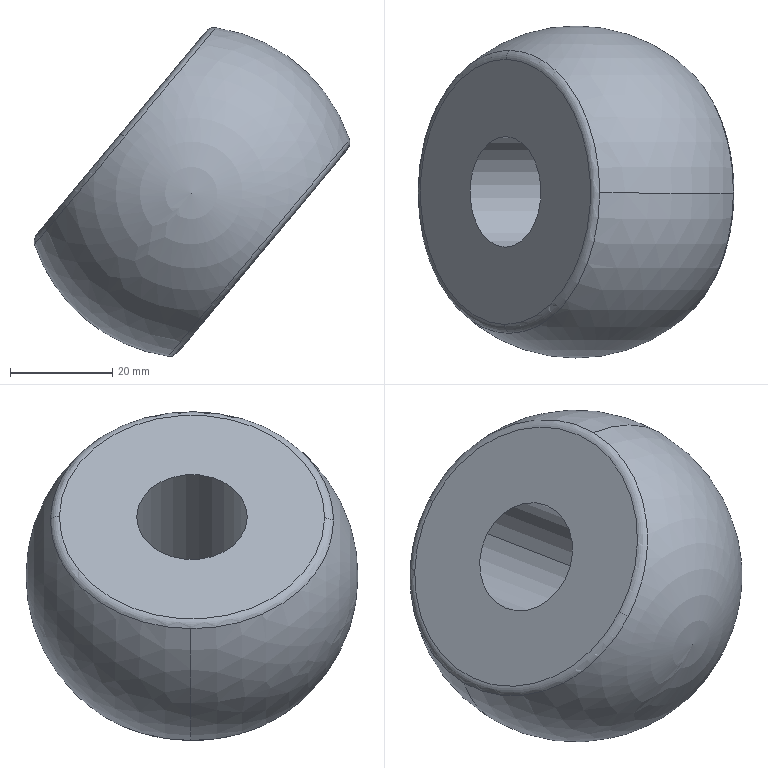Component | SolidWorks | 30-01A-1_Wheel-322-1_CJH65-322-1_CJH65wheel-322-1 | 1 solid | 10 faces | box 61.85 x 65 x 64.37 mm | volume 93907 mm3 | torus 4 | sphere 2 | cylinder 2 | plane 2 | commonest cylinder face diameters 21.667 x2
build123d program:
from build123d import *


with BuildPart() as part:
    # Sketch1 → Revolve1 (revolve)
    with BuildSketch(Plane.XY, mode=Mode.PRIVATE) as revolve1_sk:
        with BuildLine():
            Line((-18, 10.833), (18, 10.833))
            Line((18, 10.833), (18, 25.966))
            ThreePointArc((18, 25.966), (17.746, 26.941), (17.049, 27.669))
            ThreePointArc((17.049, 27.669), (0, 32.5), (-17.049, 27.669))
            ThreePointArc((-17.049, 27.669), (-17.746, 26.941), (-18, 25.966))
            Line((-18, 25.966), (-18, 10.833))
        make_face()
    revolve(revolve1_sk.sketch.rotate(Axis((50, 0, 0), (-1, 0, 0)), 270), axis=Axis((50, 0, 0), (-1, 0, 0)))


solid = part.part

# Placed as in the assembly
solid = solid.moved(Location((177.3, -622.345, -91.473), (-89.646, 0.2952, -140.136)))
STEP:
#1=CARTESIAN_POINT('',(5.767,-24.493,-4.007));
#2=VERTEX_POINT('',#1);
#3=CARTESIAN_POINT('',(6.46,-25.591,-3.178));
#4=VERTEX_POINT('',#3);
#5=CARTESIAN_POINT('',(6.465,-24.502,-3.171));
#6=DIRECTION('',(-0.7676,0.,0.641));
#7=DIRECTION('',(0.00514,1.,0.006155));
#8=AXIS2_PLACEMENT_3D('',#5,#6,#7);
#9=CIRCLE('',#8,1.089);
#10=EDGE_CURVE('',#2,#4,#9,.T.);
#11=ORIENTED_EDGE('',*,*,#10,.T.);
#12=CARTESIAN_POINT('',(6.431,-25.524,-3.153));
#13=VERTEX_POINT('',#12);
#14=CARTESIAN_POINT('',(6.492,-25.524,-3.204));
#15=DIRECTION('',(-0.641,0.008019,-0.7675));
#16=DIRECTION('',(-0.7676,0.,0.641));
#17=AXIS2_PLACEMENT_3D('',#14,#15,#16);
#18=CIRCLE('',#17,0.07874);
#19=EDGE_CURVE('',#4,#13,#18,.T.);
#20=ORIENTED_EDGE('',*,*,#19,.T.);
#21=CARTESIAN_POINT('',(6.442,-23.479,-3.141));
#22=VERTEX_POINT('',#21);
#23=CARTESIAN_POINT('',(6.436,-24.502,-3.147));
#24=DIRECTION('',(-0.7676,0.,0.641));
#25=DIRECTION('',(0.00514,1.,0.006155));
#26=AXIS2_PLACEMENT_3D('',#23,#24,#25);
#27=CIRCLE('',#26,1.022);
#28=EDGE_CURVE('',#22,#13,#27,.T.);
#29=ORIENTED_EDGE('',*,*,#28,.F.);
#30=CARTESIAN_POINT('',(6.471,-23.412,-3.164));
#31=VERTEX_POINT('',#30);
#32=CARTESIAN_POINT('',(6.502,-23.479,-3.191));
#33=DIRECTION('',(0.641,-0.008019,0.7675));
#34=DIRECTION('',(0.7676,0.,-0.641));
#35=AXIS2_PLACEMENT_3D('',#32,#33,#34);
#36=CIRCLE('',#35,0.07874);
#37=EDGE_CURVE('',#31,#22,#36,.T.);
#38=ORIENTED_EDGE('',*,*,#37,.F.);
#39=CARTESIAN_POINT('',(6.465,-24.502,-3.171));
#40=DIRECTION('',(-0.7676,0.,0.641));
#41=DIRECTION('',(0.00514,1.,0.006155));
#42=AXIS2_PLACEMENT_3D('',#39,#40,#41);
#43=CIRCLE('',#42,1.089);
#44=EDGE_CURVE('',#31,#2,#43,.T.);
#45=ORIENTED_EDGE('',*,*,#44,.T.);
#46=EDGE_LOOP('',(#11,#20,#29,#38,#45));
#47=FACE_OUTER_BOUND('',#46,.T.);
#48=CARTESIAN_POINT('',(6.497,-24.502,-3.198));
#49=DIRECTION('',(-0.7676,0.,0.641));
#50=DIRECTION('',(0.00514,1.,0.006155));
#51=AXIS2_PLACEMENT_3D('',#48,#49,#50);
#52=TOROIDAL_SURFACE('',#51,1.022,0.07874);
#53=ADVANCED_FACE('',(#47),#52,.T.);
#54=CARTESIAN_POINT('',(7.49,-25.591,-4.038));
#55=VERTEX_POINT('',#54);
#56=CARTESIAN_POINT('',(8.194,-24.51,-3.195));
#57=VERTEX_POINT('',#56);
#58=CARTESIAN_POINT('',(7.496,-24.502,-4.032));
#59=DIRECTION('',(-0.7676,0.,0.641));
#60=DIRECTION('',(0.00514,1.,0.006155));
#61=AXIS2_PLACEMENT_3D('',#58,#59,#60);
#62=CIRCLE('',#61,1.089);
#63=EDGE_CURVE('',#55,#57,#62,.T.);
#64=ORIENTED_EDGE('',*,*,#63,.T.);
#65=CARTESIAN_POINT('',(7.163,-24.51,-2.335));
#66=VERTEX_POINT('',#65);
#67=CARTESIAN_POINT('',(6.98,-24.502,-3.601));
#68=DIRECTION('',(-0.00514,-1.,-0.006155));
#69=DIRECTION('',(0.,0.006155,-1.));
#70=AXIS2_PLACEMENT_3D('',#67,#68,#69);
#71=CIRCLE('',#70,1.28);
#72=EDGE_CURVE('',#57,#66,#71,.T.);
#73=ORIENTED_EDGE('',*,*,#72,.T.);
#74=CARTESIAN_POINT('',(6.465,-24.502,-3.171));
#75=DIRECTION('',(-0.7676,0.,0.641));
#76=DIRECTION('',(0.00514,1.,0.006155));
#77=AXIS2_PLACEMENT_3D('',#74,#75,#76);
#78=CIRCLE('',#77,1.089);
#79=EDGE_CURVE('',#4,#66,#78,.T.);
#80=ORIENTED_EDGE('',*,*,#79,.F.);
#81=ORIENTED_EDGE('',*,*,#10,.F.);
#82=CARTESIAN_POINT('',(6.797,-24.493,-4.868));
#83=VERTEX_POINT('',#82);
#84=CARTESIAN_POINT('',(6.98,-24.502,-3.601));
#85=DIRECTION('',(0.00514,1.,0.006155));
#86=DIRECTION('',(0.,-0.006155,1.));
#87=AXIS2_PLACEMENT_3D('',#84,#85,#86);
#88=CIRCLE('',#87,1.28);
#89=EDGE_CURVE('',#83,#2,#88,.T.);
#90=ORIENTED_EDGE('',*,*,#89,.F.);
#91=CARTESIAN_POINT('',(7.496,-24.502,-4.032));
#92=DIRECTION('',(-0.7676,0.,0.641));
#93=DIRECTION('',(0.00514,1.,0.006155));
#94=AXIS2_PLACEMENT_3D('',#91,#92,#93);
#95=CIRCLE('',#94,1.089);
#96=EDGE_CURVE('',#83,#55,#95,.T.);
#97=ORIENTED_EDGE('',*,*,#96,.T.);
#98=EDGE_LOOP('',(#64,#73,#80,#81,#90,#97));
#99=FACE_OUTER_BOUND('',#98,.T.);
#100=CARTESIAN_POINT('',(6.98,-24.502,-3.601));
#101=DIRECTION('',(-0.00514,-1.,-0.006155));
#102=DIRECTION('',(-0.641,0.008019,-0.7675));
#103=AXIS2_PLACEMENT_3D('',#100,#101,#102);
#104=SPHERICAL_SURFACE('',#103,1.28);
#105=ADVANCED_FACE('',(#99),#104,.T.);
#106=CARTESIAN_POINT('',(7.529,-23.479,-4.049));
#107=VERTEX_POINT('',#106);
#108=CARTESIAN_POINT('',(7.519,-25.524,-4.062));
#109=VERTEX_POINT('',#108);
#110=CARTESIAN_POINT('',(7.524,-24.502,-4.056));
#111=DIRECTION('',(-0.7676,0.,0.641));
#112=DIRECTION('',(0.00514,1.,0.006155));
#113=AXIS2_PLACEMENT_3D('',#110,#111,#112);
#114=CIRCLE('',#113,1.022);
#115=EDGE_CURVE('',#107,#109,#114,.T.);
#116=ORIENTED_EDGE('',*,*,#115,.T.);
#117=CARTESIAN_POINT('',(7.459,-25.524,-4.011));
#118=DIRECTION('',(-0.641,0.008019,-0.7675));
#119=DIRECTION('',(-0.7676,0.,0.641));
#120=AXIS2_PLACEMENT_3D('',#117,#118,#119);
#121=CIRCLE('',#120,0.07874);
#122=EDGE_CURVE('',#109,#55,#121,.T.);
#123=ORIENTED_EDGE('',*,*,#122,.T.);
#124=ORIENTED_EDGE('',*,*,#96,.F.);
#125=CARTESIAN_POINT('',(7.501,-23.412,-4.025));
#126=VERTEX_POINT('',#125);
#127=CARTESIAN_POINT('',(7.496,-24.502,-4.032));
#128=DIRECTION('',(-0.7676,0.,0.641));
#129=DIRECTION('',(0.00514,1.,0.006155));
#130=AXIS2_PLACEMENT_3D('',#127,#128,#129);
#131=CIRCLE('',#130,1.089);
#132=EDGE_CURVE('',#126,#83,#131,.T.);
#133=ORIENTED_EDGE('',*,*,#132,.F.);
#134=CARTESIAN_POINT('',(7.469,-23.479,-3.999));
#135=DIRECTION('',(0.641,-0.008019,0.7675));
#136=DIRECTION('',(0.7676,0.,-0.641));
#137=AXIS2_PLACEMENT_3D('',#134,#135,#136);
#138=CIRCLE('',#137,0.07874);
#139=EDGE_CURVE('',#107,#126,#138,.T.);
#140=ORIENTED_EDGE('',*,*,#139,.F.);
#141=EDGE_LOOP('',(#116,#123,#124,#133,#140));
#142=FACE_OUTER_BOUND('',#141,.T.);
#143=CARTESIAN_POINT('',(7.464,-24.502,-4.005));
#144=DIRECTION('',(-0.7676,0.,0.641));
#145=DIRECTION('',(0.00514,1.,0.006155));
#146=AXIS2_PLACEMENT_3D('',#143,#144,#145);
#147=TOROIDAL_SURFACE('',#146,1.022,0.07874);
#148=ADVANCED_FACE('',(#142),#147,.T.);
#149=CARTESIAN_POINT('',(7.522,-24.928,-4.058));
#150=VERTEX_POINT('',#149);
#151=CARTESIAN_POINT('',(7.526,-24.075,-4.053));
#152=VERTEX_POINT('',#151);
#153=CARTESIAN_POINT('',(7.524,-24.502,-4.056));
#154=DIRECTION('',(-0.7676,0.,0.641));
#155=DIRECTION('',(0.00514,1.,0.006155));
#156=AXIS2_PLACEMENT_3D('',#153,#154,#155);
#157=CIRCLE('',#156,0.4265);
#158=EDGE_CURVE('',#150,#152,#157,.T.);
#159=ORIENTED_EDGE('',*,*,#158,.F.);
#160=CARTESIAN_POINT('',(6.434,-24.928,-3.15));
#161=VERTEX_POINT('',#160);
#162=CARTESIAN_POINT('',(8.489,-24.928,-4.866));
#163=DIRECTION('',(-0.7676,0.,0.641));
#164=VECTOR('',#163,39.37);
#165=LINE('',#162,#164);
#166=EDGE_CURVE('',#150,#161,#165,.T.);
#167=ORIENTED_EDGE('',*,*,#166,.T.);
#168=CARTESIAN_POINT('',(6.439,-24.075,-3.144));
#169=VERTEX_POINT('',#168);
#170=CARTESIAN_POINT('',(6.436,-24.502,-3.147));
#171=DIRECTION('',(-0.7676,0.,0.641));
#172=DIRECTION('',(0.00514,1.,0.006155));
#173=AXIS2_PLACEMENT_3D('',#170,#171,#172);
#174=CIRCLE('',#173,0.4265);
#175=EDGE_CURVE('',#161,#169,#174,.T.);
#176=ORIENTED_EDGE('',*,*,#175,.T.);
#177=CARTESIAN_POINT('',(8.493,-24.075,-4.86));
#178=DIRECTION('',(-0.7676,0.,0.641));
#179=VECTOR('',#178,39.37);
#180=LINE('',#177,#179);
#181=EDGE_CURVE('',#152,#169,#180,.T.);
#182=ORIENTED_EDGE('',*,*,#181,.F.);
#183=EDGE_LOOP('',(#159,#167,#176,#182));
#184=FACE_OUTER_BOUND('',#183,.T.);
#185=CARTESIAN_POINT('',(8.491,-24.502,-4.863));
#186=DIRECTION('',(-0.7676,0.,0.641));
#187=DIRECTION('',(0.00514,1.,0.006155));
#188=AXIS2_PLACEMENT_3D('',#185,#186,#187);
#189=CYLINDRICAL_SURFACE('',#188,0.4265);
#190=ADVANCED_FACE('',(#184),#189,.F.);
#191=CARTESIAN_POINT('',(6.436,-24.502,-3.147));
#192=DIRECTION('',(-0.7676,0.,0.641));
#193=DIRECTION('',(0.00514,1.,0.006155));
#194=AXIS2_PLACEMENT_3D('',#191,#192,#193);
#195=CIRCLE('',#194,0.4265);
#196=EDGE_CURVE('',#169,#161,#195,.T.);
#197=ORIENTED_EDGE('',*,*,#196,.F.);
#198=ORIENTED_EDGE('',*,*,#175,.F.);
#199=EDGE_LOOP('',(#197,#198));
#200=FACE_BOUND('',#199,.T.);
#201=ORIENTED_EDGE('',*,*,#28,.T.);
#202=CARTESIAN_POINT('',(6.436,-24.502,-3.147));
#203=DIRECTION('',(-0.7676,0.,0.641));
#204=DIRECTION('',(0.00514,1.,0.006155));
#205=AXIS2_PLACEMENT_3D('',#202,#203,#204);
#206=CIRCLE('',#205,1.022);
#207=EDGE_CURVE('',#13,#22,#206,.T.);
#208=ORIENTED_EDGE('',*,*,#207,.T.);
#209=EDGE_LOOP('',(#201,#208));
#210=FACE_OUTER_BOUND('',#209,.T.);
#211=CARTESIAN_POINT('',(5.781,-24.494,-3.932));
#212=DIRECTION('',(0.7676,-0.,-0.641));
#213=DIRECTION('',(-0.00514,-1.,-0.006155));
#214=AXIS2_PLACEMENT_3D('',#211,#212,#213);
#215=PLANE('',#214);
#216=ADVANCED_FACE('',(#200,#210),#215,.F.);
#217=ORIENTED_EDGE('',*,*,#166,.F.);
#218=CARTESIAN_POINT('',(7.524,-24.502,-4.056));
#219=DIRECTION('',(-0.7676,0.,0.641));
#220=DIRECTION('',(0.00514,1.,0.006155));
#221=AXIS2_PLACEMENT_3D('',#218,#219,#220);
#222=CIRCLE('',#221,0.4265);
#223=EDGE_CURVE('',#152,#150,#222,.T.);
#224=ORIENTED_EDGE('',*,*,#223,.F.);
#225=ORIENTED_EDGE('',*,*,#181,.T.);
#226=ORIENTED_EDGE('',*,*,#196,.T.);
#227=EDGE_LOOP('',(#217,#224,#225,#226));
#228=FACE_OUTER_BOUND('',#227,.T.);
#229=CARTESIAN_POINT('',(8.491,-24.502,-4.863));
#230=DIRECTION('',(-0.7676,0.,0.641));
#231=DIRECTION('',(0.00514,1.,0.006155));
#232=AXIS2_PLACEMENT_3D('',#229,#230,#231);
#233=CYLINDRICAL_SURFACE('',#232,0.4265);
#234=ADVANCED_FACE('',(#228),#233,.F.);
#235=ORIENTED_EDGE('',*,*,#115,.F.);
#236=CARTESIAN_POINT('',(7.524,-24.502,-4.056));
#237=DIRECTION('',(-0.7676,0.,0.641));
#238=DIRECTION('',(0.00514,1.,0.006155));
#239=AXIS2_PLACEMENT_3D('',#236,#237,#238);
#240=CIRCLE('',#239,1.022);
#241=EDGE_CURVE('',#109,#107,#240,.T.);
#242=ORIENTED_EDGE('',*,*,#241,.F.);
#243=EDGE_LOOP('',(#235,#242));
#244=FACE_OUTER_BOUND('',#243,.T.);
#245=ORIENTED_EDGE('',*,*,#223,.T.);
#246=ORIENTED_EDGE('',*,*,#158,.T.);
#247=EDGE_LOOP('',(#245,#246));
#248=FACE_BOUND('',#247,.T.);
#249=CARTESIAN_POINT('',(7.251,-24.498,-4.383));
#250=DIRECTION('',(-0.7676,0.,0.641));
#251=DIRECTION('',(0.00514,1.,0.006155));
#252=AXIS2_PLACEMENT_3D('',#249,#250,#251);
#253=PLANE('',#252);
#254=ADVANCED_FACE('',(#244,#248),#253,.F.);
#255=ORIENTED_EDGE('',*,*,#122,.F.);
#256=ORIENTED_EDGE('',*,*,#241,.T.);
#257=ORIENTED_EDGE('',*,*,#139,.T.);
#258=CARTESIAN_POINT('',(7.496,-24.502,-4.032));
#259=DIRECTION('',(-0.7676,0.,0.641));
#260=DIRECTION('',(0.00514,1.,0.006155));
#261=AXIS2_PLACEMENT_3D('',#258,#259,#260);
#262=CIRCLE('',#261,1.089);
#263=EDGE_CURVE('',#57,#126,#262,.T.);
#264=ORIENTED_EDGE('',*,*,#263,.F.);
#265=ORIENTED_EDGE('',*,*,#63,.F.);
#266=EDGE_LOOP('',(#255,#256,#257,#264,#265));
#267=FACE_OUTER_BOUND('',#266,.T.);
#268=CARTESIAN_POINT('',(7.464,-24.502,-4.005));
#269=DIRECTION('',(-0.7676,0.,0.641));
#270=DIRECTION('',(0.00514,1.,0.006155));
#271=AXIS2_PLACEMENT_3D('',#268,#269,#270);
#272=TOROIDAL_SURFACE('',#271,1.022,0.07874);
#273=ADVANCED_FACE('',(#267),#272,.T.);
#274=ORIENTED_EDGE('',*,*,#72,.F.);
#275=ORIENTED_EDGE('',*,*,#263,.T.);
#276=ORIENTED_EDGE('',*,*,#132,.T.);
#277=ORIENTED_EDGE('',*,*,#89,.T.);
#278=ORIENTED_EDGE('',*,*,#44,.F.);
#279=CARTESIAN_POINT('',(6.465,-24.502,-3.171));
#280=DIRECTION('',(-0.7676,0.,0.641));
#281=DIRECTION('',(0.00514,1.,0.006155));
#282=AXIS2_PLACEMENT_3D('',#279,#280,#281);
#283=CIRCLE('',#282,1.089);
#284=EDGE_CURVE('',#66,#31,#283,.T.);
#285=ORIENTED_EDGE('',*,*,#284,.F.);
#286=EDGE_LOOP('',(#274,#275,#276,#277,#278,#285));
#287=FACE_OUTER_BOUND('',#286,.T.);
#288=CARTESIAN_POINT('',(6.98,-24.502,-3.601));
#289=DIRECTION('',(-0.00514,-1.,-0.006155));
#290=DIRECTION('',(-0.641,0.008019,-0.7675));
#291=AXIS2_PLACEMENT_3D('',#288,#289,#290);
#292=SPHERICAL_SURFACE('',#291,1.28);
#293=ADVANCED_FACE('',(#287),#292,.T.);
#294=ORIENTED_EDGE('',*,*,#19,.F.);
#295=ORIENTED_EDGE('',*,*,#79,.T.);
#296=ORIENTED_EDGE('',*,*,#284,.T.);
#297=ORIENTED_EDGE('',*,*,#37,.T.);
#298=ORIENTED_EDGE('',*,*,#207,.F.);
#299=EDGE_LOOP('',(#294,#295,#296,#297,#298));
#300=FACE_OUTER_BOUND('',#299,.T.);
#301=CARTESIAN_POINT('',(6.497,-24.502,-3.198));
#302=DIRECTION('',(-0.7676,0.,0.641));
#303=DIRECTION('',(0.00514,1.,0.006155));
#304=AXIS2_PLACEMENT_3D('',#301,#302,#303);
#305=TOROIDAL_SURFACE('',#304,1.022,0.07874);
#306=ADVANCED_FACE('',(#300),#305,.T.);
#307=CLOSED_SHELL('',(#53,#105,#148,#190,#216,#234,#254,#273,#293,#306));
#308=MANIFOLD_SOLID_BREP('',#307);
#309=CARTESIAN_POINT('',(0.,0.,0.));
#310=DIRECTION('',(0.,0.,1.));
#311=DIRECTION('',(1.,0.,0.));
#312=AXIS2_PLACEMENT_3D('',#309,#310,#311);
#313=(LENGTH_UNIT()NAMED_UNIT(*)SI_UNIT($,.METRE.));
#314=LENGTH_MEASURE_WITH_UNIT(LENGTH_MEASURE(0.0254),#313);
#315=DIMENSIONAL_EXPONENTS(1.,0.,0.,0.,0.,0.,0.);
#316=(CONVERSION_BASED_UNIT('',#314)LENGTH_UNIT()NAMED_UNIT(#315));
#317=UNCERTAINTY_MEASURE_WITH_UNIT(LENGTH_MEASURE(0.00001),#316,'','');
#318=(NAMED_UNIT(*)PLANE_ANGLE_UNIT()SI_UNIT($,.RADIAN.));
#319=(NAMED_UNIT(*)SI_UNIT($,.STERADIAN.)SOLID_ANGLE_UNIT());
#320=(GEOMETRIC_REPRESENTATION_CONTEXT(3)GLOBAL_UNCERTAINTY_ASSIGNED_CONTEXT((#317))GLOBAL_UNIT_ASSIGNED_CONTEXT((#316,#318,#319))REPRESENTATION_CONTEXT('',''));
#321=ADVANCED_BREP_SHAPE_REPRESENTATION('',(#308,#312),#320);
#322=COLOUR_RGB('',0.7922,0.8196,0.9333);
#323=FILL_AREA_STYLE_COLOUR('',#322);
#324=FILL_AREA_STYLE('',(#323));
#325=SURFACE_STYLE_FILL_AREA(#324);
#326=SURFACE_SIDE_STYLE('',(#325));
#327=SURFACE_STYLE_USAGE(.BOTH.,#326);
#328=PRESENTATION_STYLE_ASSIGNMENT((#327));
#329=STYLED_ITEM('',(#328),#308);
#330=PRESENTATION_LAYER_ASSIGNMENT('','',(#329));
#331=(LENGTH_UNIT()NAMED_UNIT(*)SI_UNIT($,.METRE.));
#332=LENGTH_MEASURE_WITH_UNIT(LENGTH_MEASURE(0.0254),#331);
#333=DIMENSIONAL_EXPONENTS(1.,0.,0.,0.,0.,0.,0.);
#334=(CONVERSION_BASED_UNIT('',#332)LENGTH_UNIT()NAMED_UNIT(#333));
#335=UNCERTAINTY_MEASURE_WITH_UNIT(LENGTH_MEASURE(0.00001),#334,'','');
#336=(NAMED_UNIT(*)PLANE_ANGLE_UNIT()SI_UNIT($,.RADIAN.));
#337=(NAMED_UNIT(*)SI_UNIT($,.STERADIAN.)SOLID_ANGLE_UNIT());
#338=(GEOMETRIC_REPRESENTATION_CONTEXT(3)GLOBAL_UNCERTAINTY_ASSIGNED_CONTEXT((#335))GLOBAL_UNIT_ASSIGNED_CONTEXT((#334,#336,#337))REPRESENTATION_CONTEXT('',''));
#339=MECHANICAL_DESIGN_GEOMETRIC_PRESENTATION_REPRESENTATION('',(#329),#338);